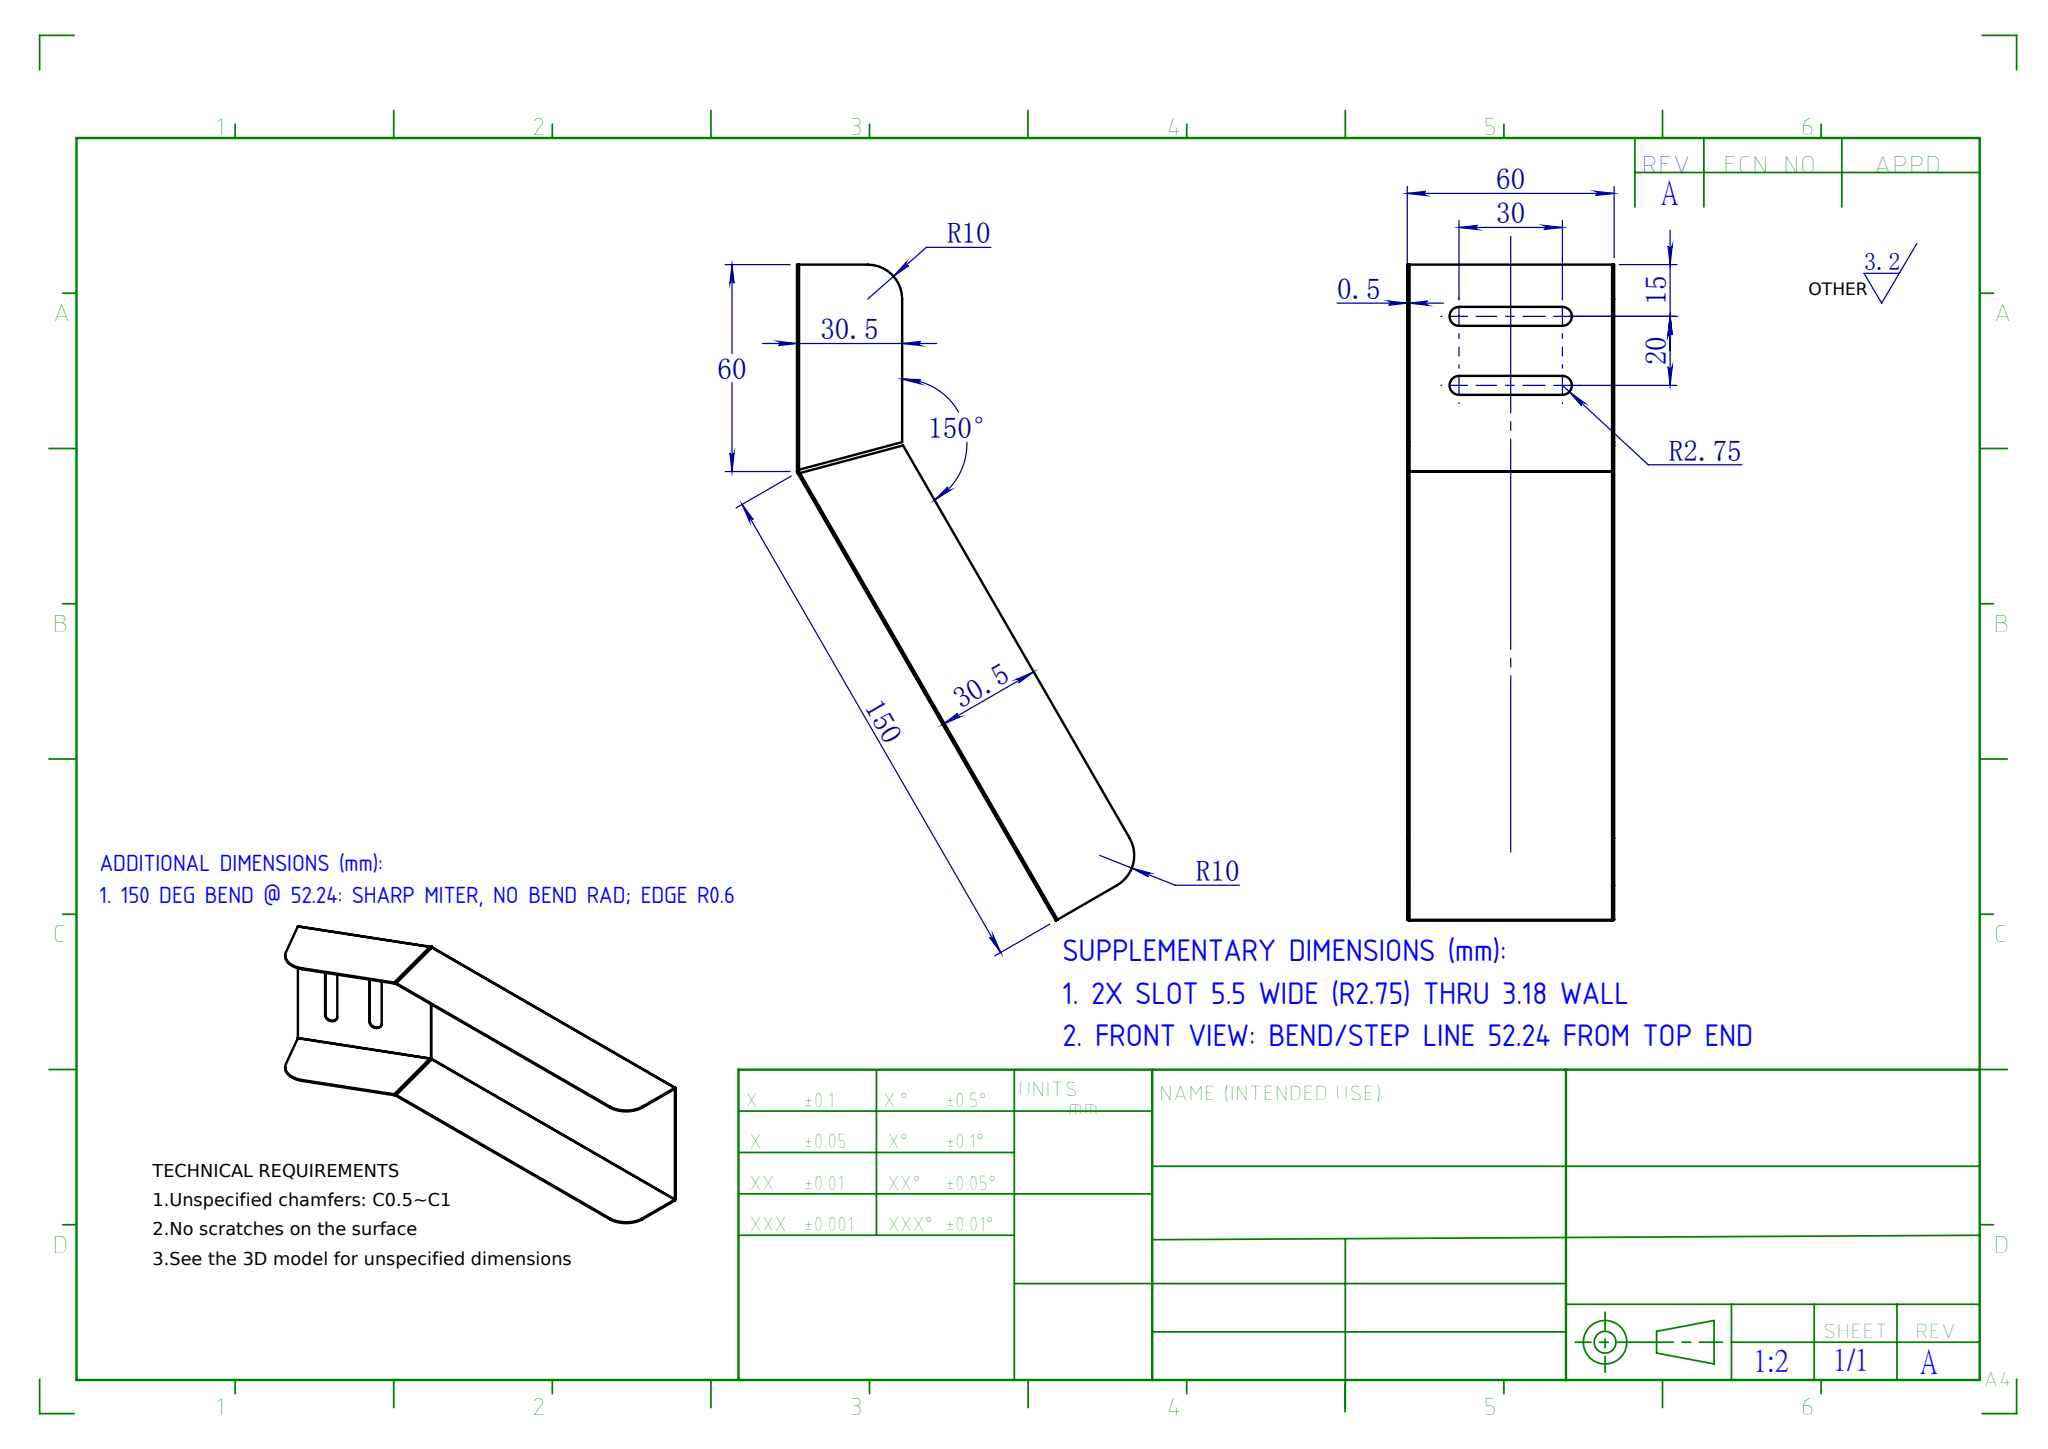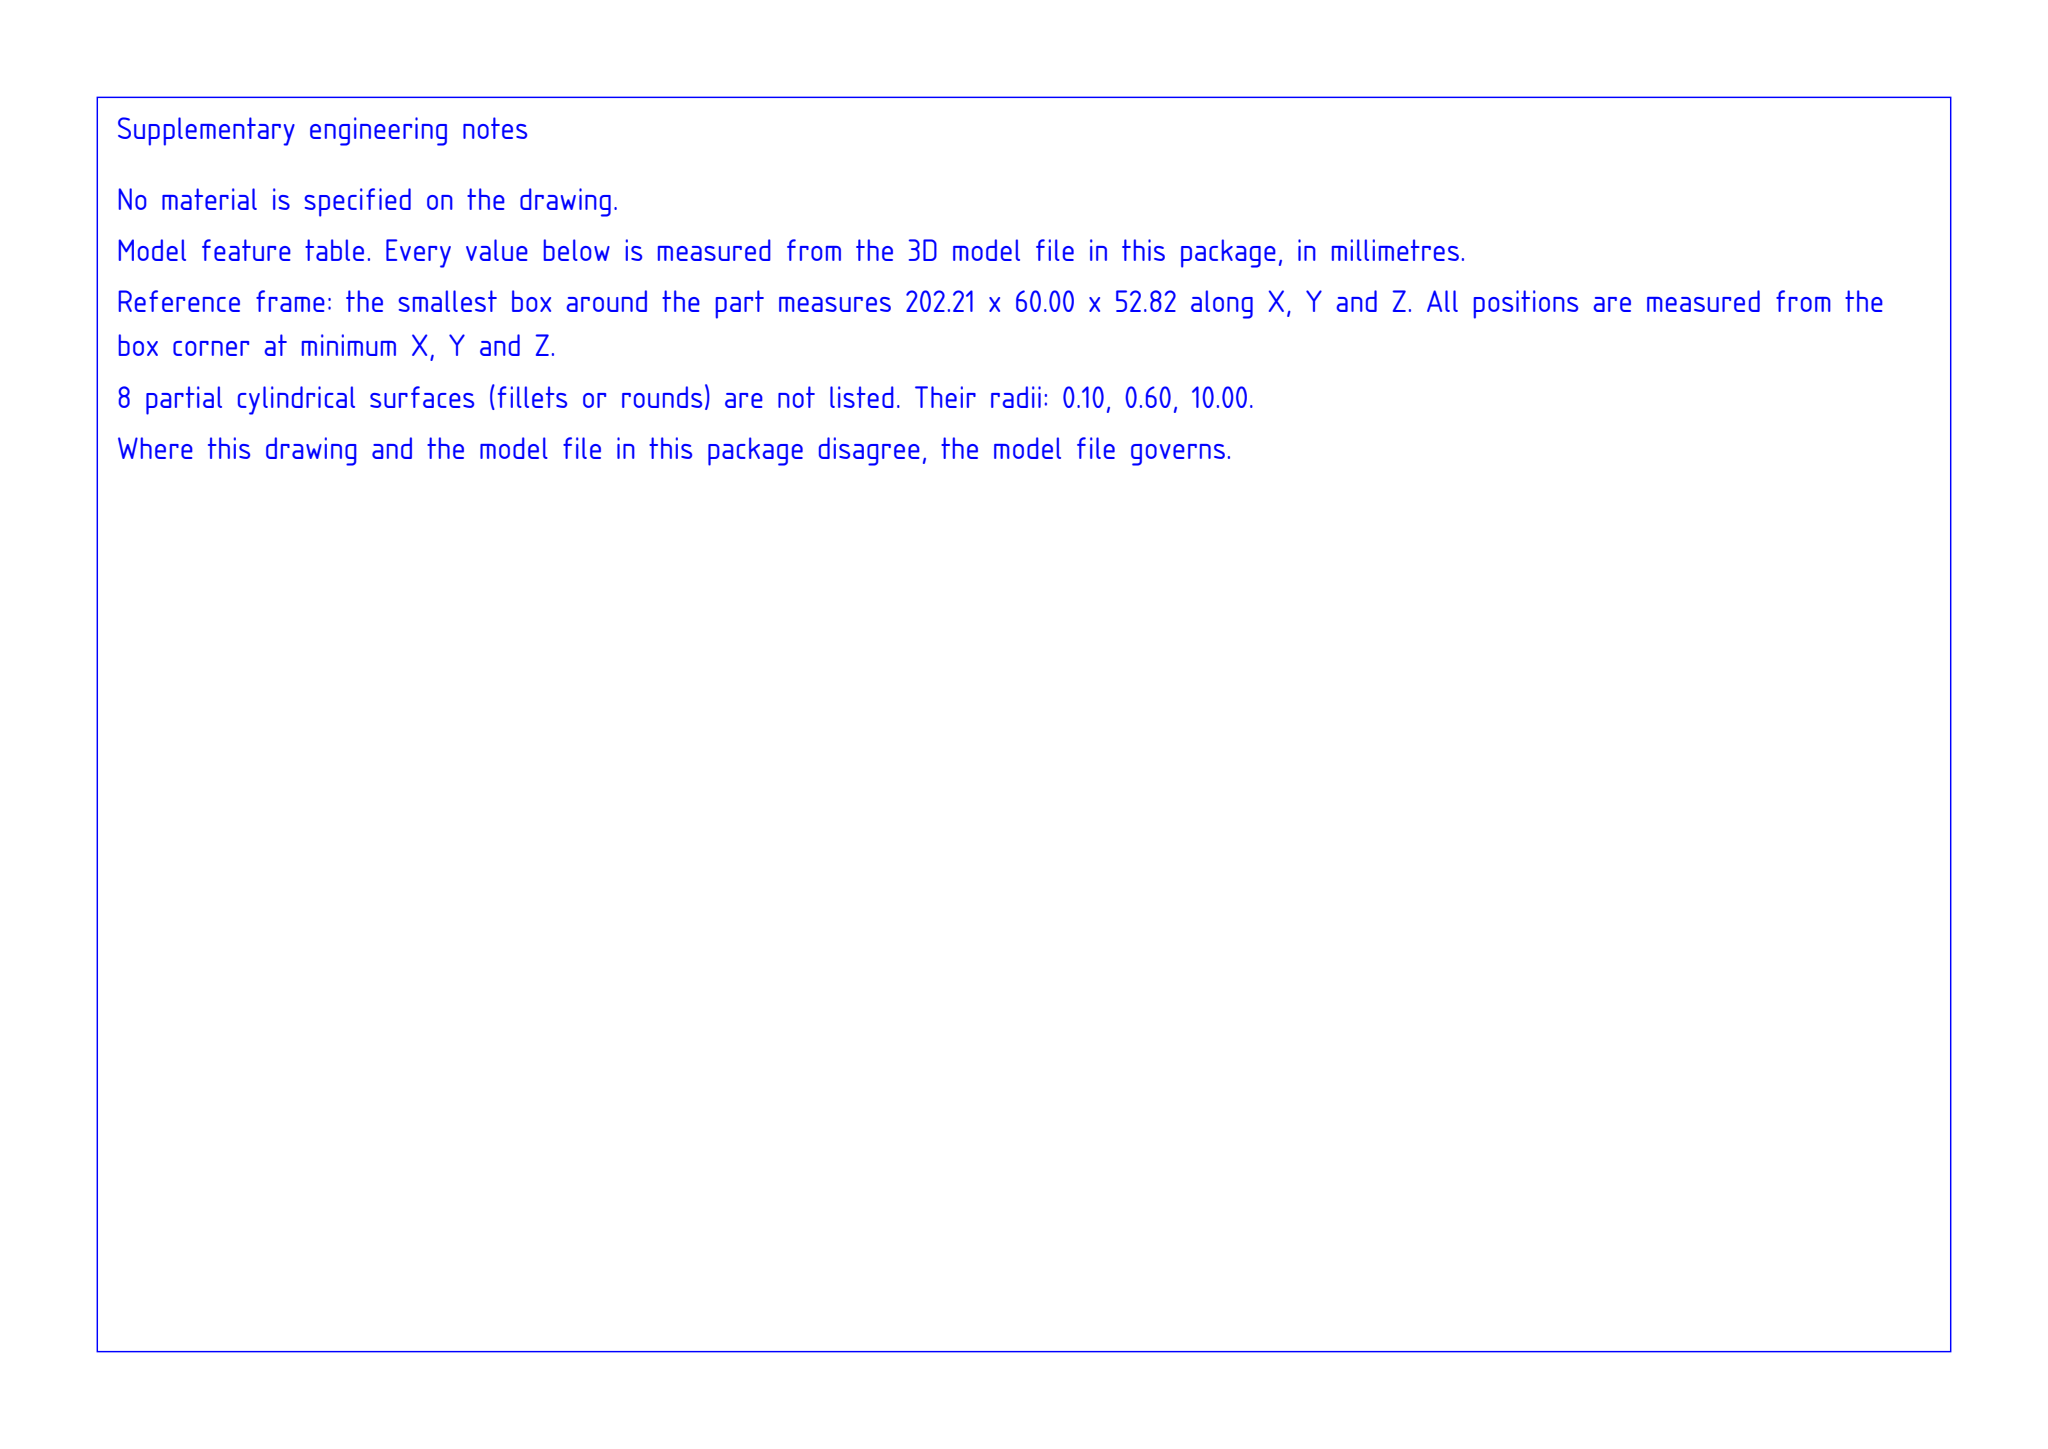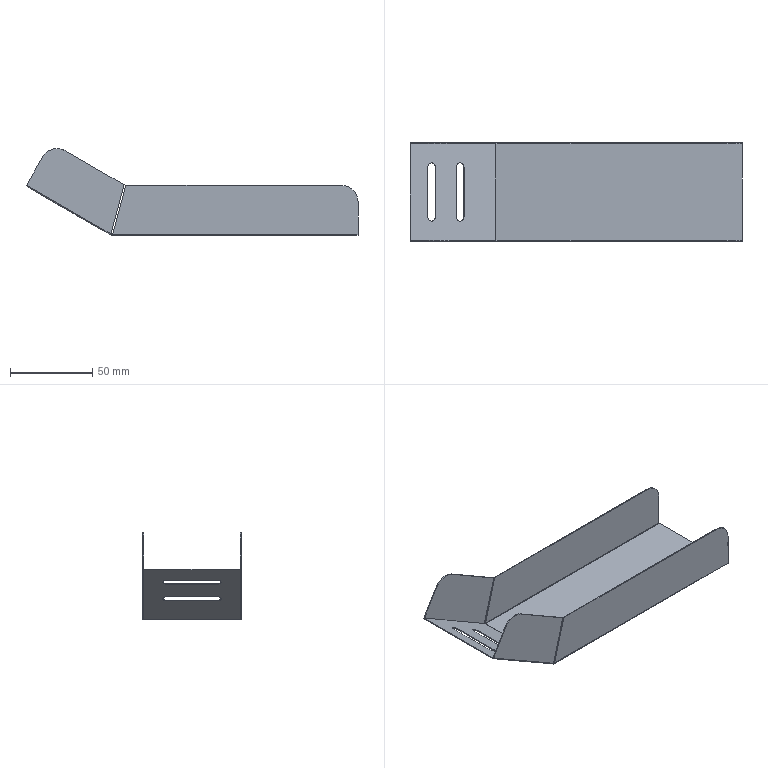Part | SolidWorks | mm | 1 solid | 63 faces | box 202.21 x 60 x 52.82 mm | volume 12068 mm3 | plane 40 | cylinder 19 | spline 4 | commonest cylinder face diameters 20 x5 1.2 x5 0.2 x5 5.5 x4